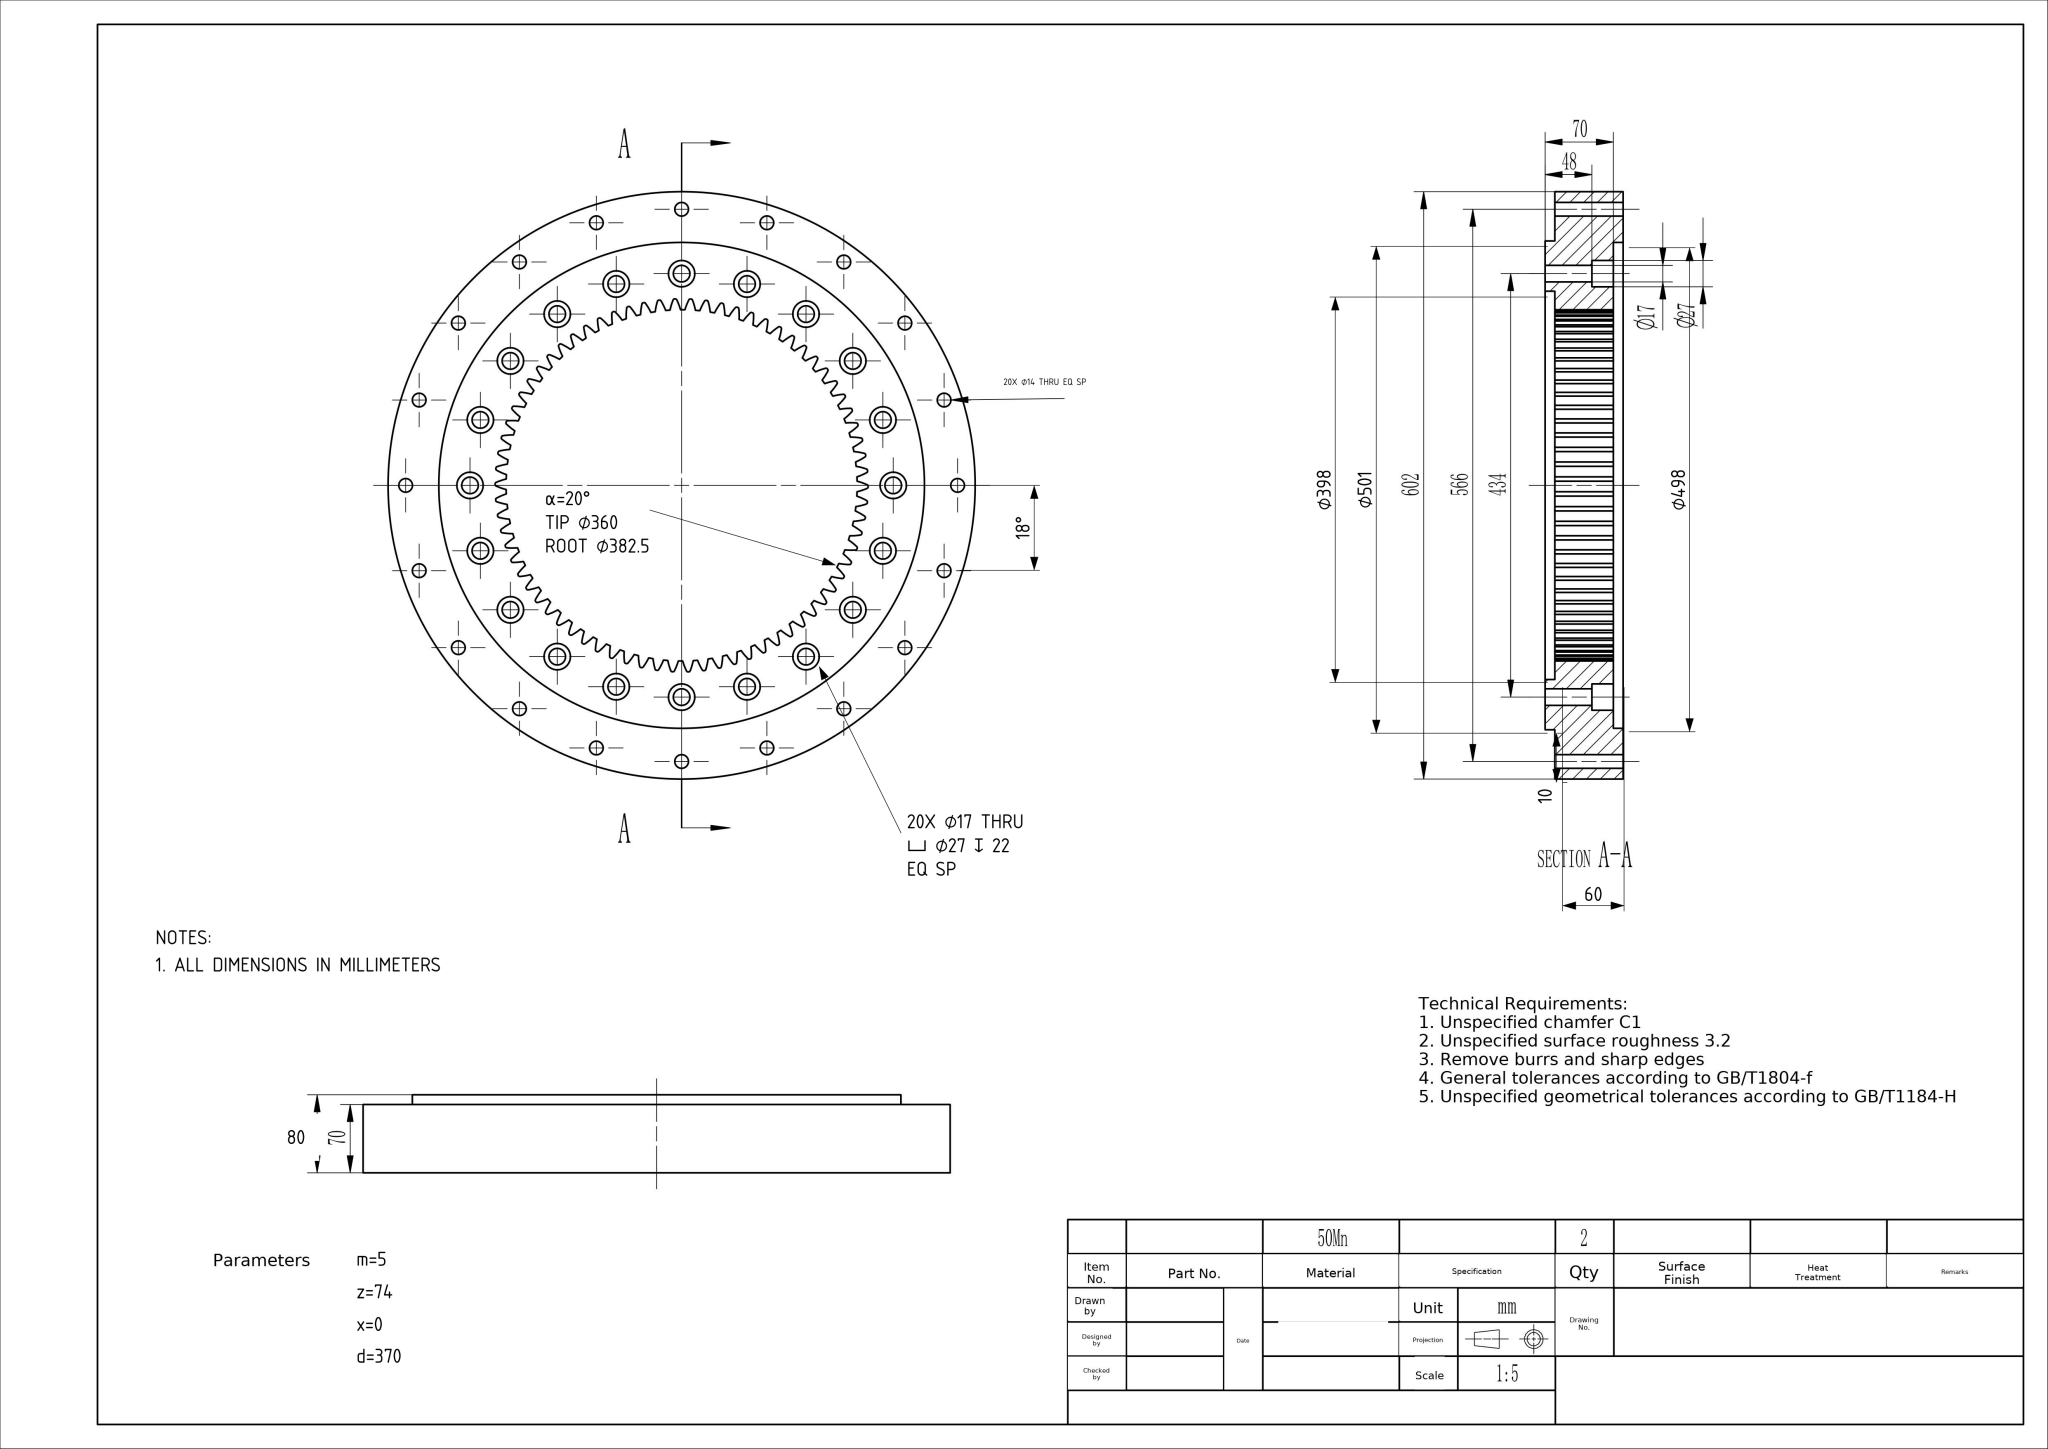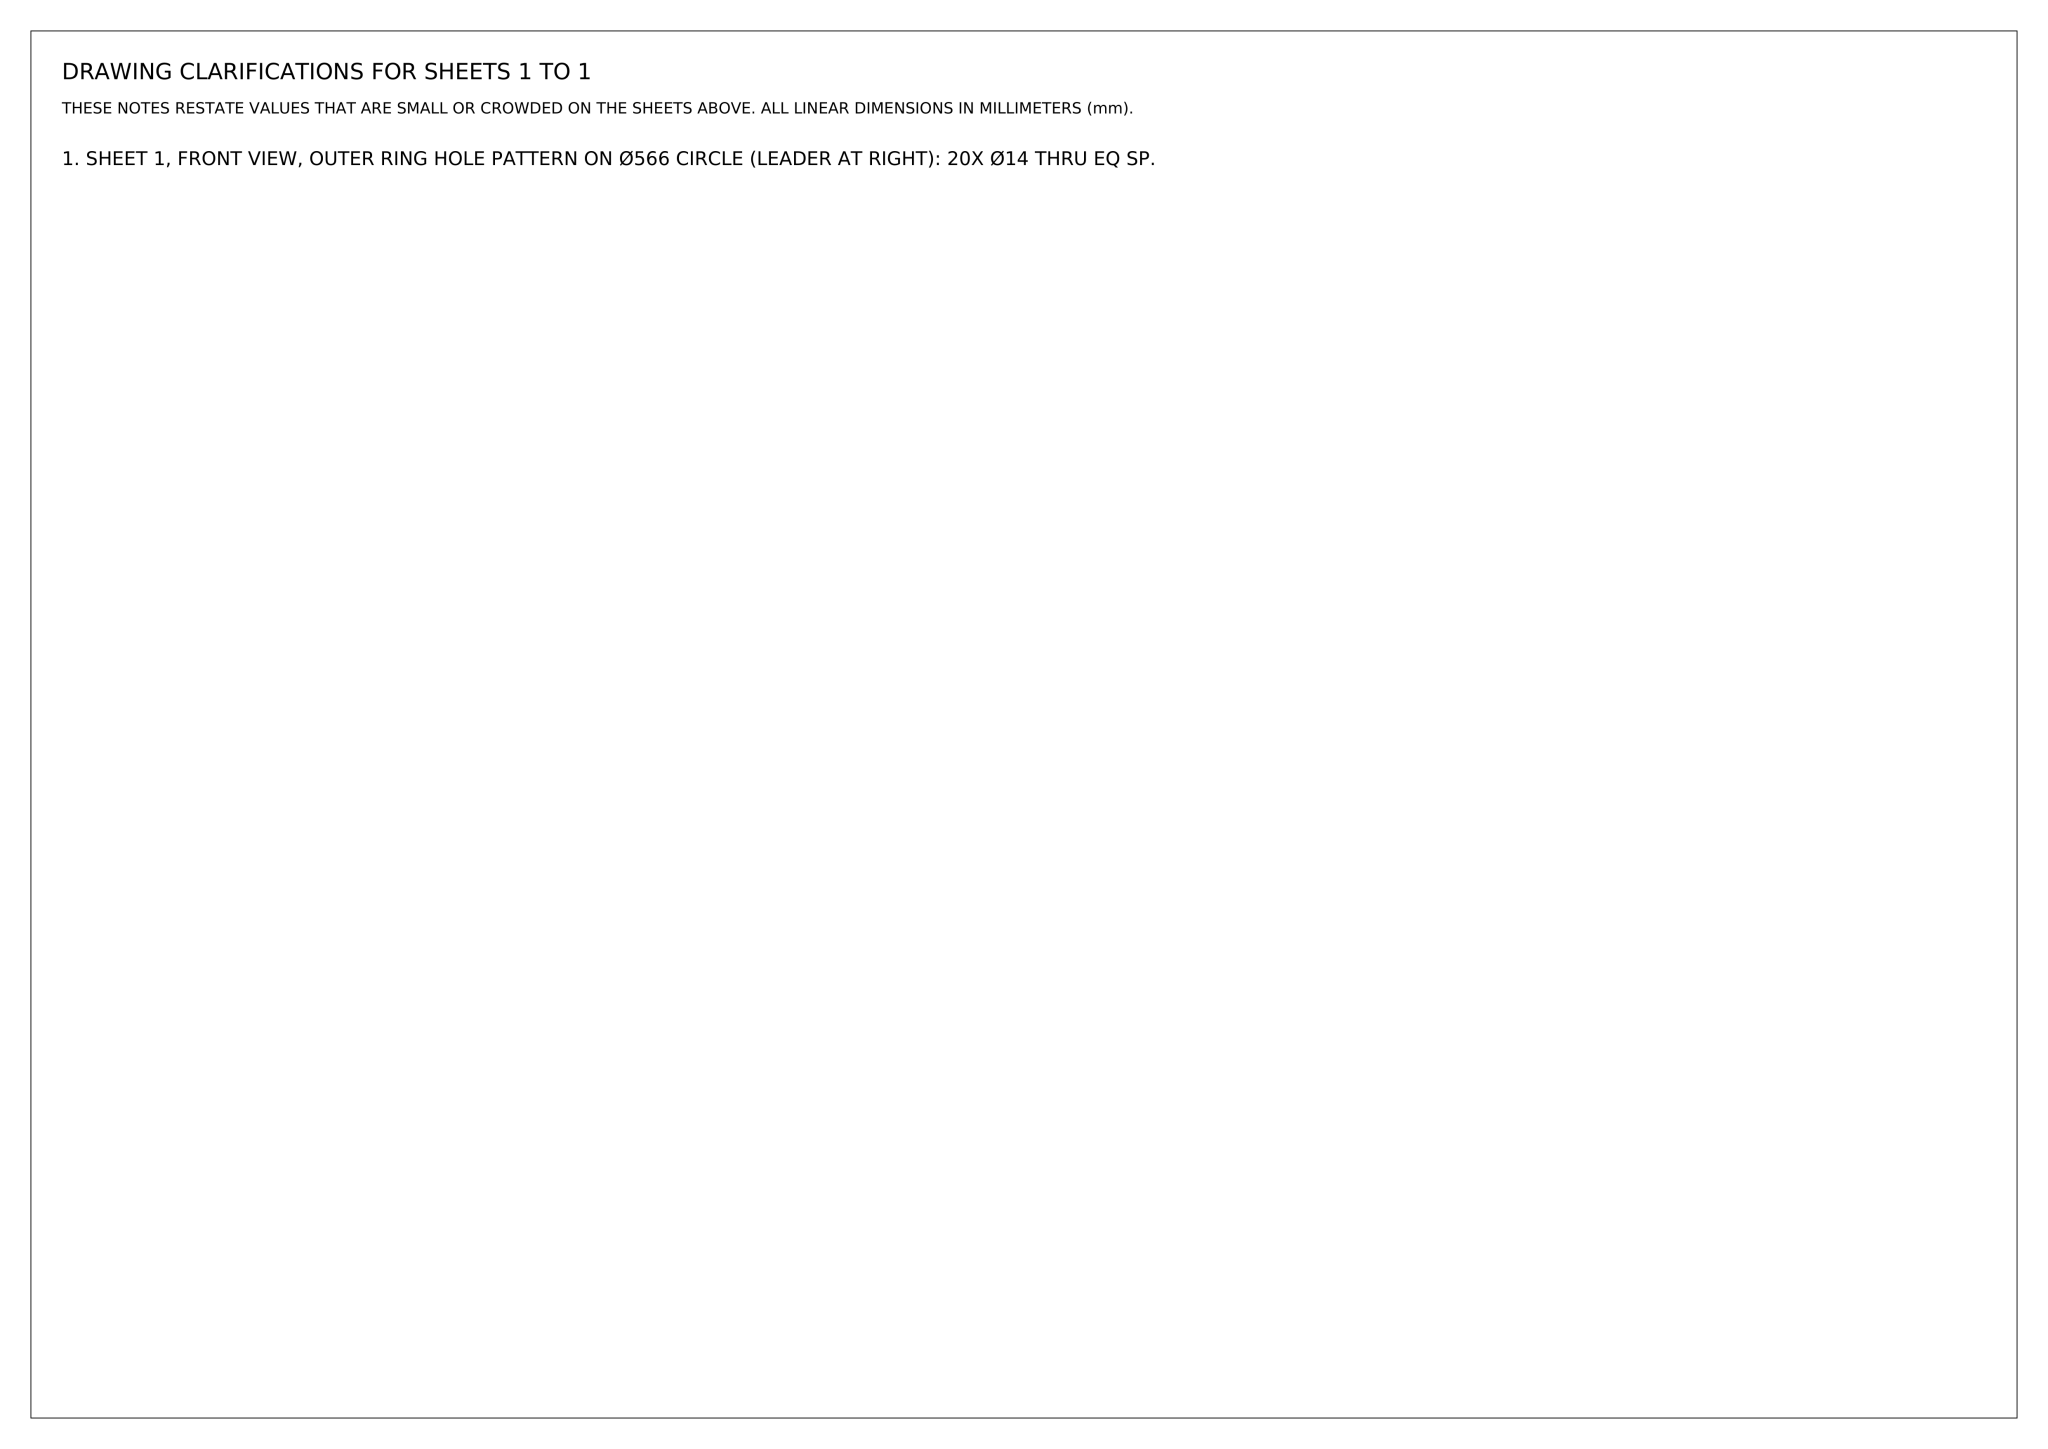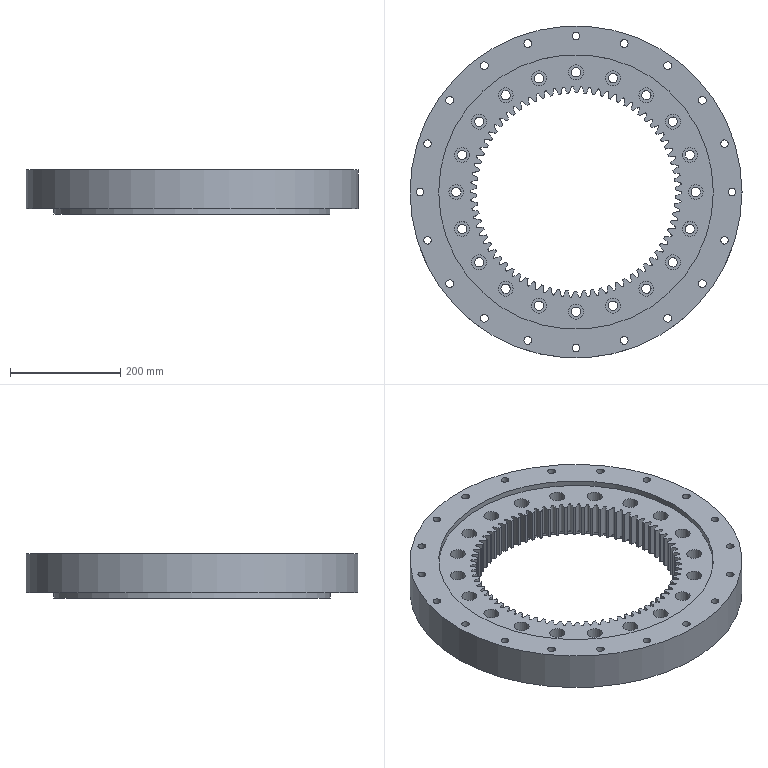Part | NX | mm | 1 solid | 237 faces | box 602 x 602 x 80 mm | volume 12013969 mm3 | cylinder 138 | spline 74 | plane 25 | commonest cylinder face diameters 360 x74 17 x20 14 x20 27 x20 602 x1 501 x1 398 x1 498 x1